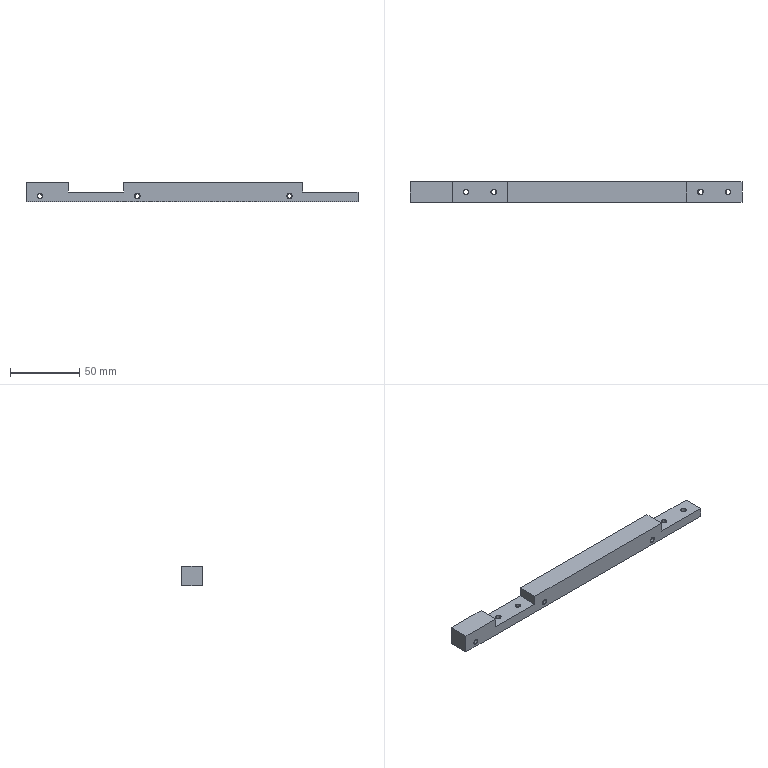CAM job | Mastercam | mm | 13 operations | part box 240 x 15 x 14
1. Facing | 24 - 50 平铣刀
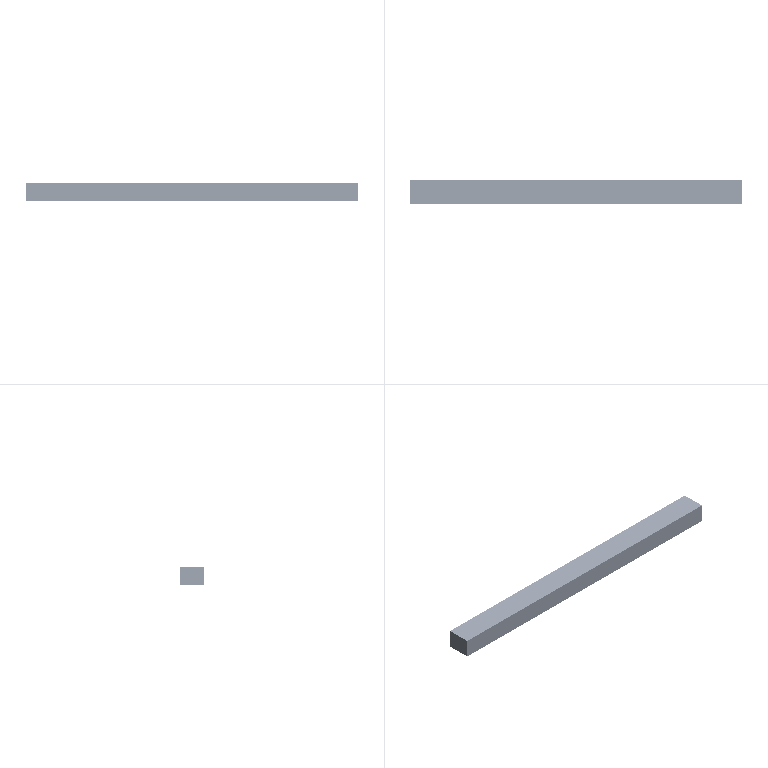2. Contour (Ramp) | 10 - 10 平铣刀
3. Contour (2D) | 8 - 8 平铣刀
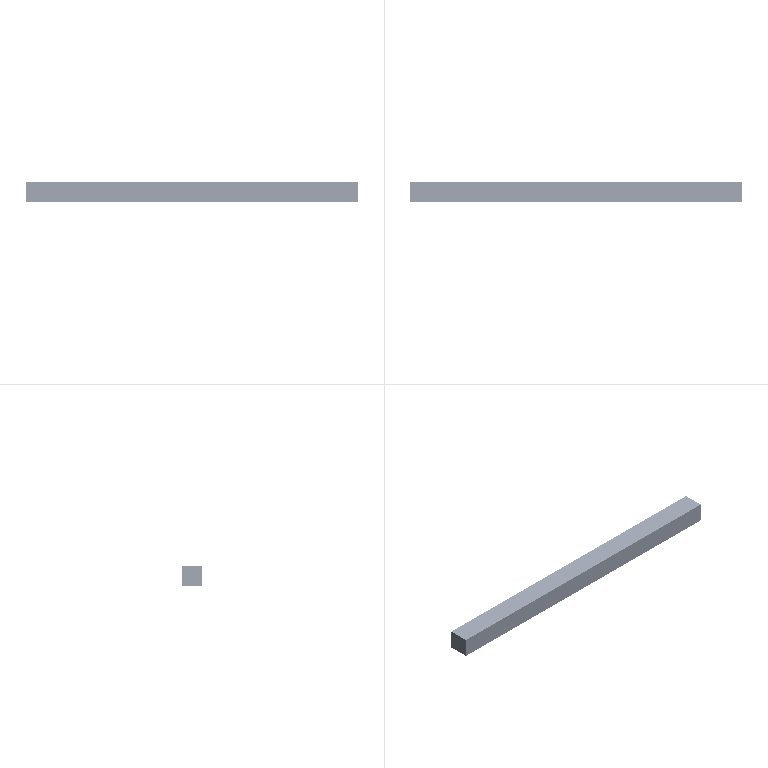4. Contour (2D chamfer) | 7 - 4 倒角刀
5. Facing | 24 - 50 平铣刀
6. Contour (Ramp) | 10 - 10 平铣刀
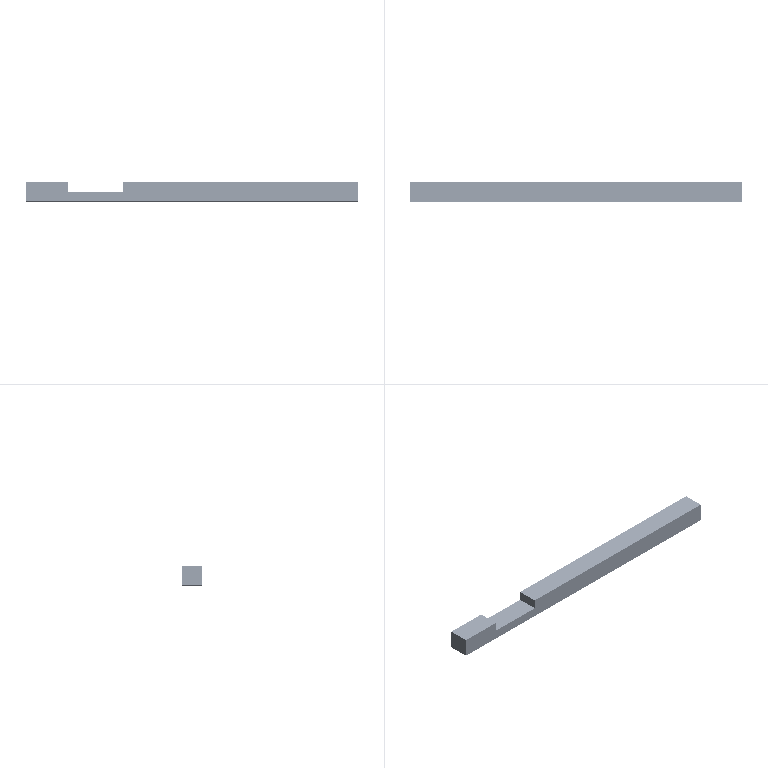7. Contour (2D) | 10 - 10 平铣刀
8. Contour (Ramp) | 10 - 10 平铣刀
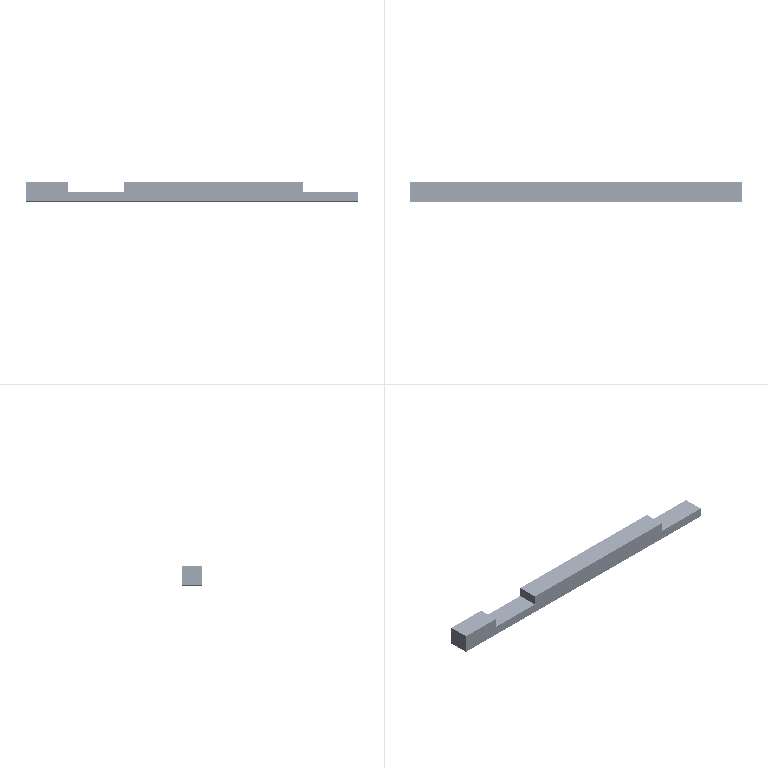9. Contour (2D) | 10 - 10 平铣刀
10. Contour (2D chamfer) | 7 - 4 倒角刀
11. Contour (2D chamfer) | 7 - 4 倒角刀
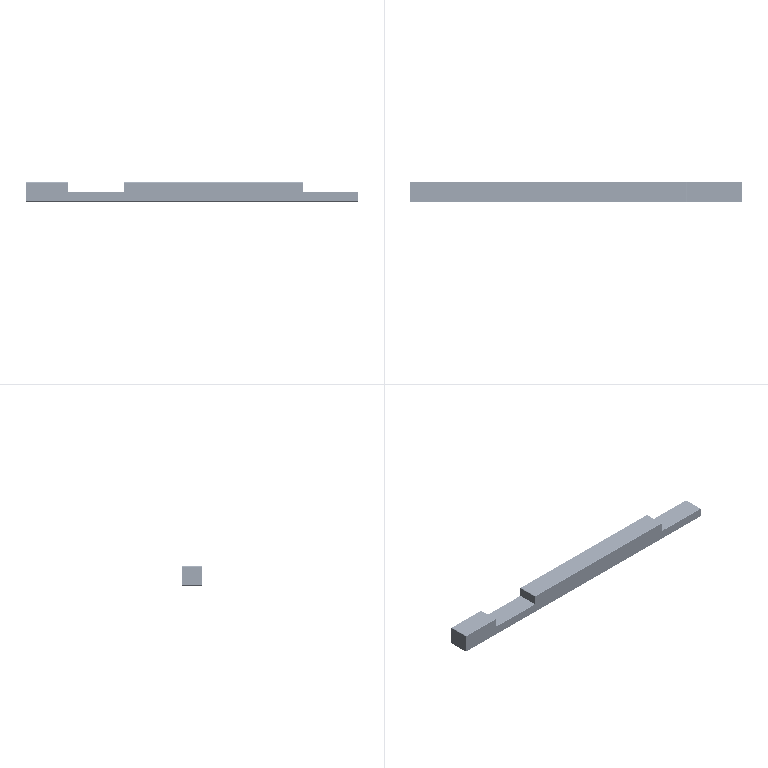12. Drill/Counterbore | 7 - 4 倒角刀
13. Drill/Counterbore | 7 - 4 倒角刀